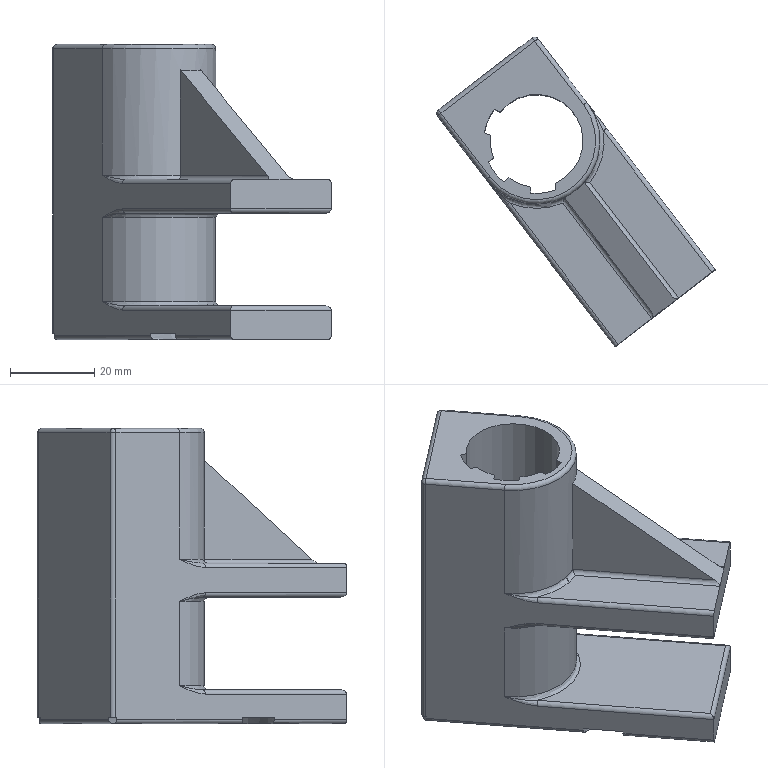Component | NX | CA6140-ZHOU12-BOCHA1 | 1 solid | 71 faces | volume 58781 mm3 | cylinder 32 | plane 24 | spline 6 | torus 5 | sphere 4 | commonest cylinder face diameters 2 x20 22 x3 25 x3 48 x3 30 x2 64 x1